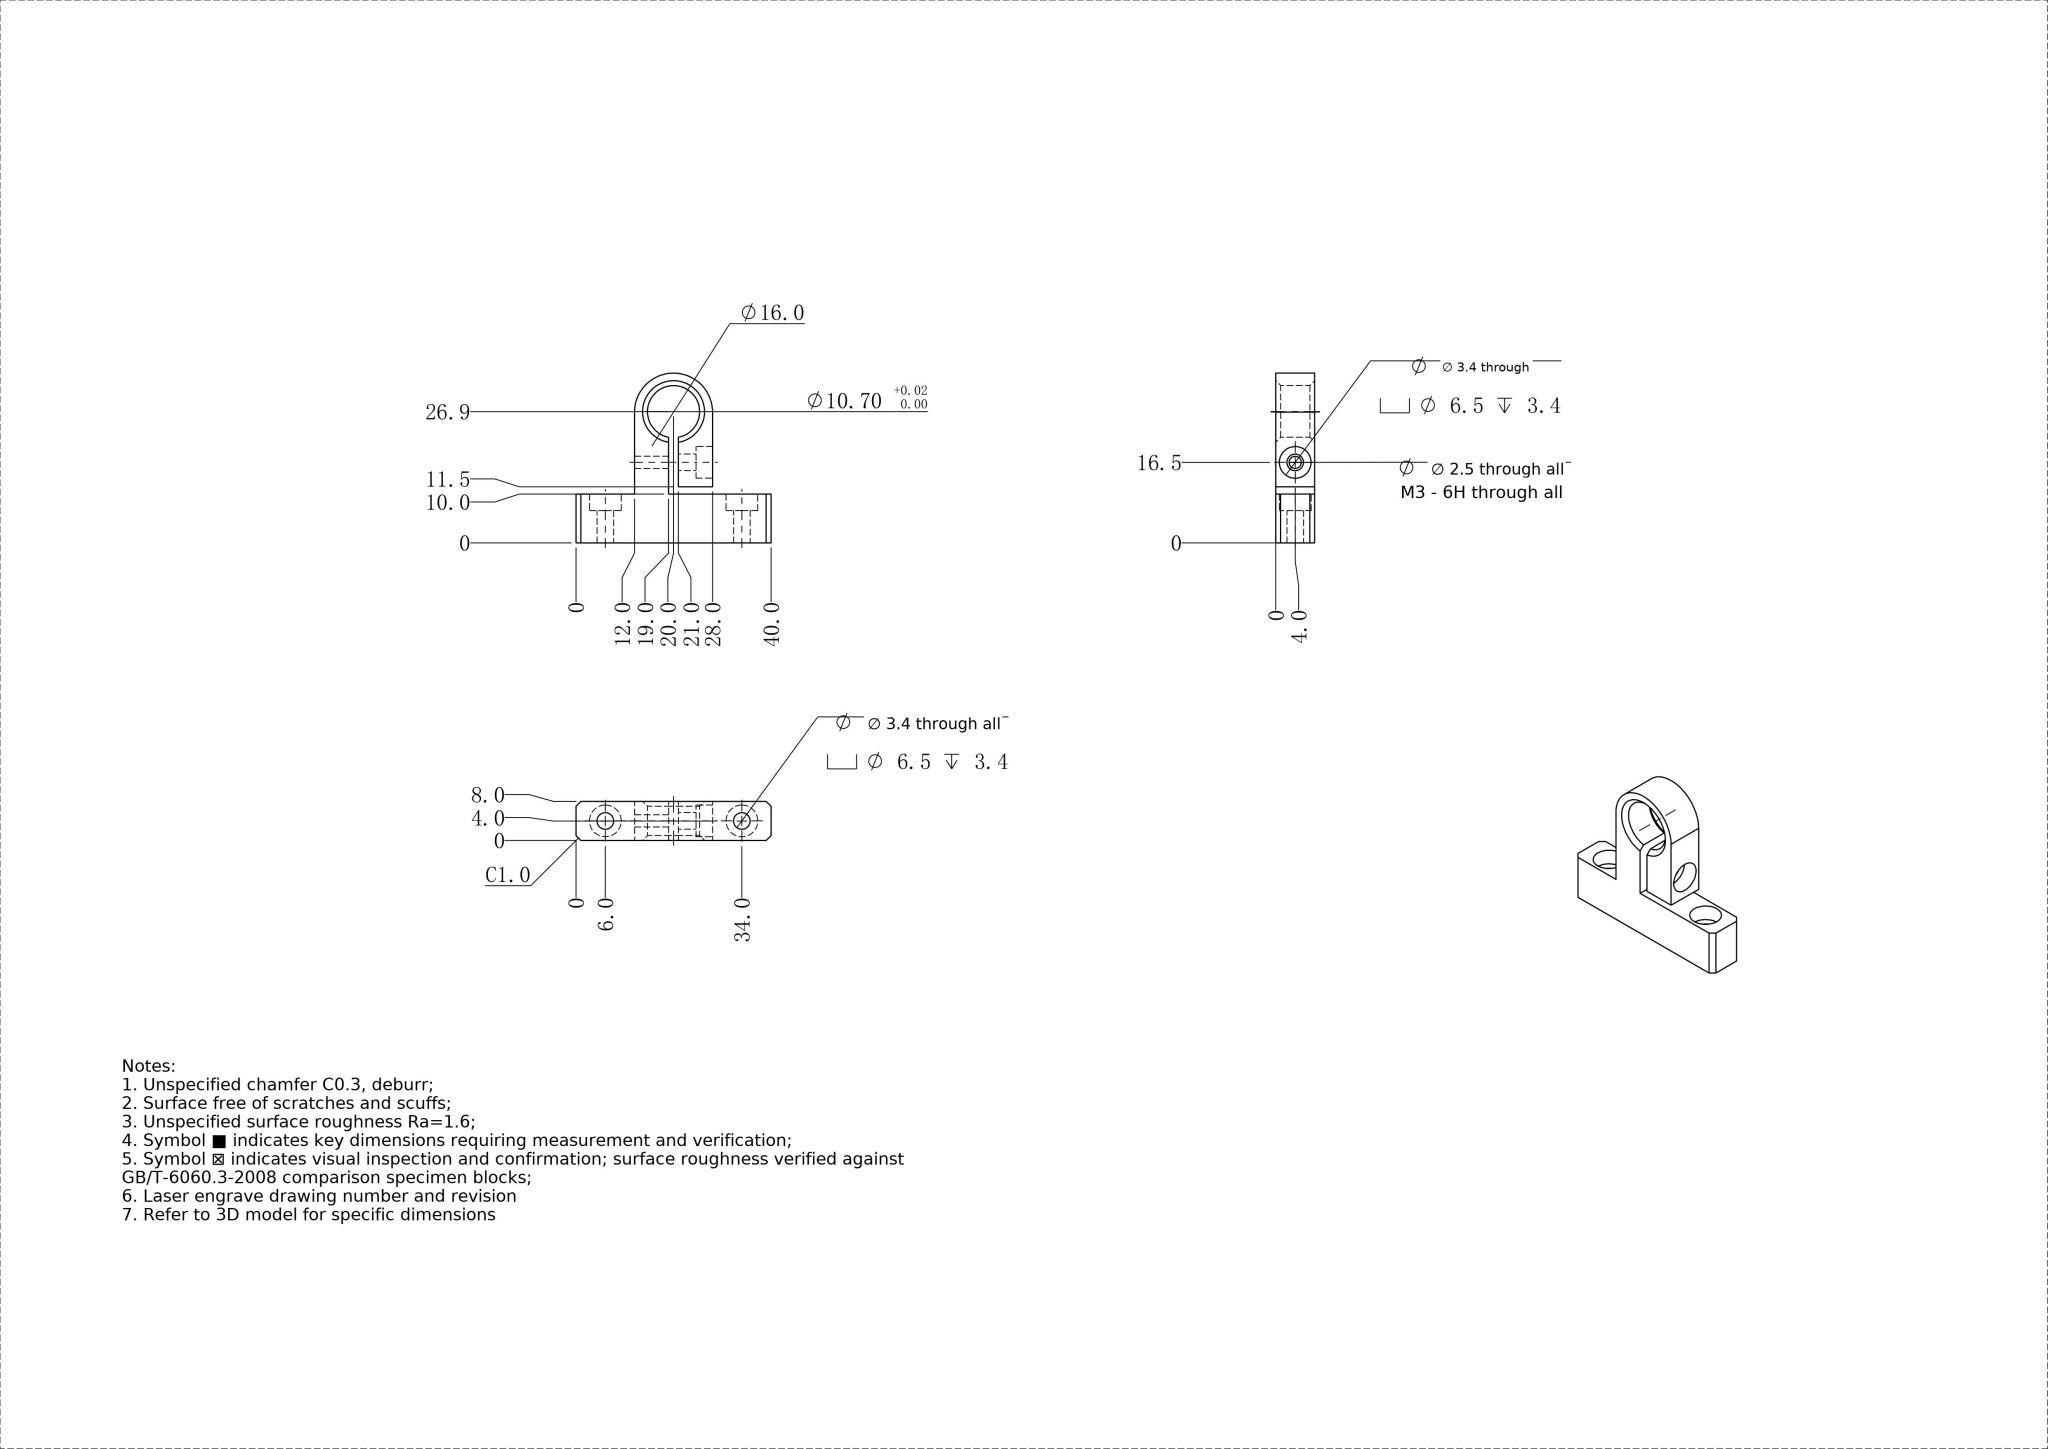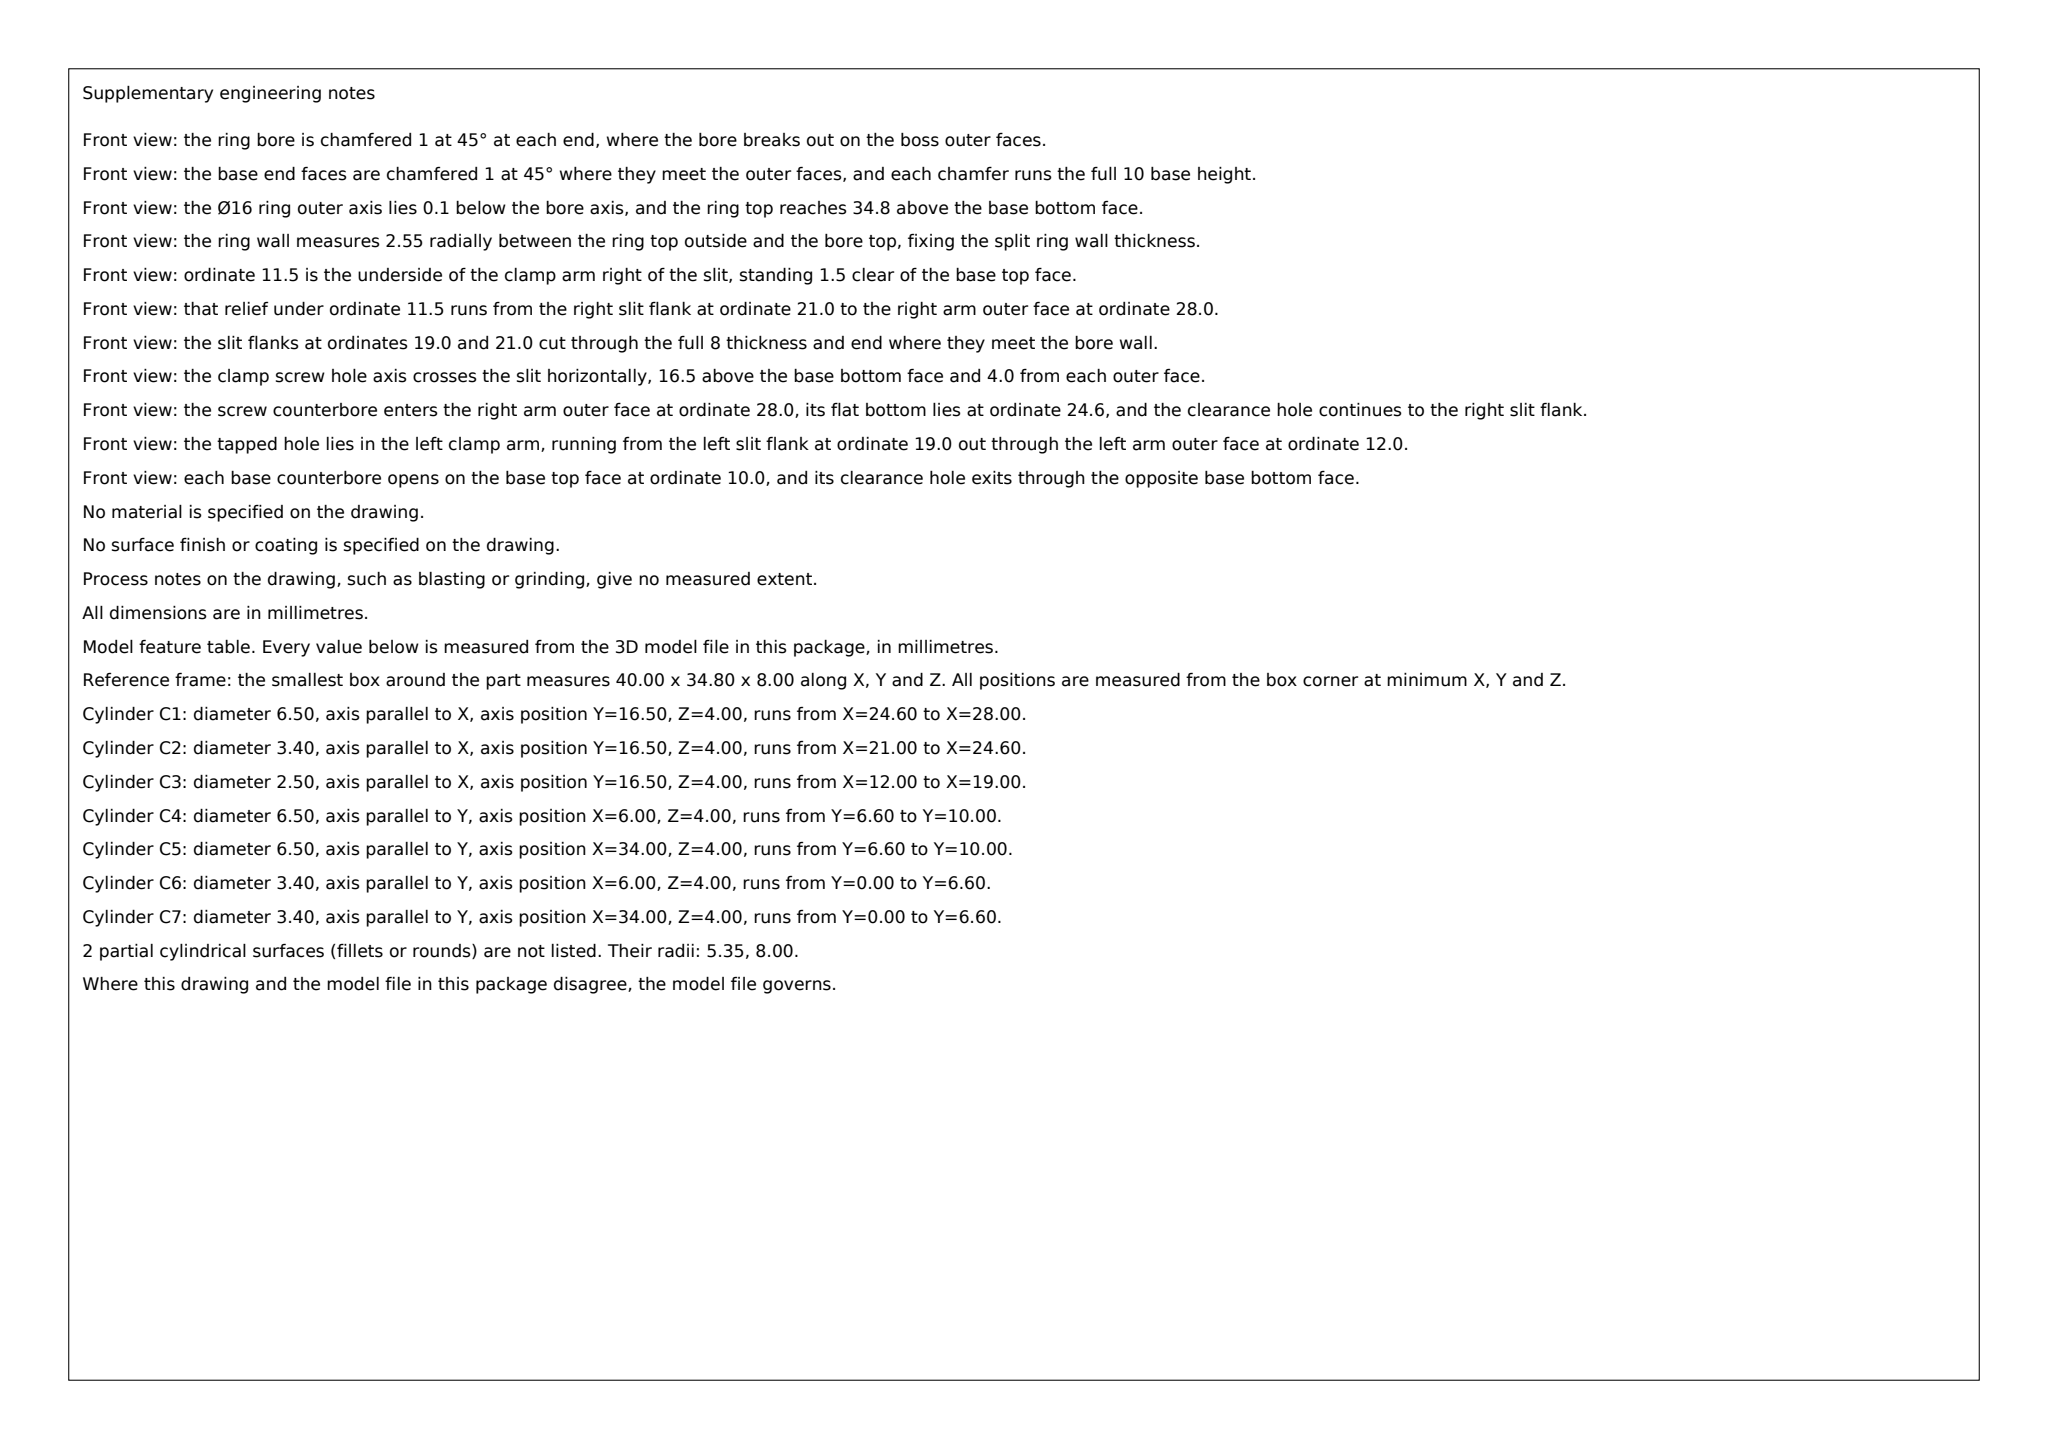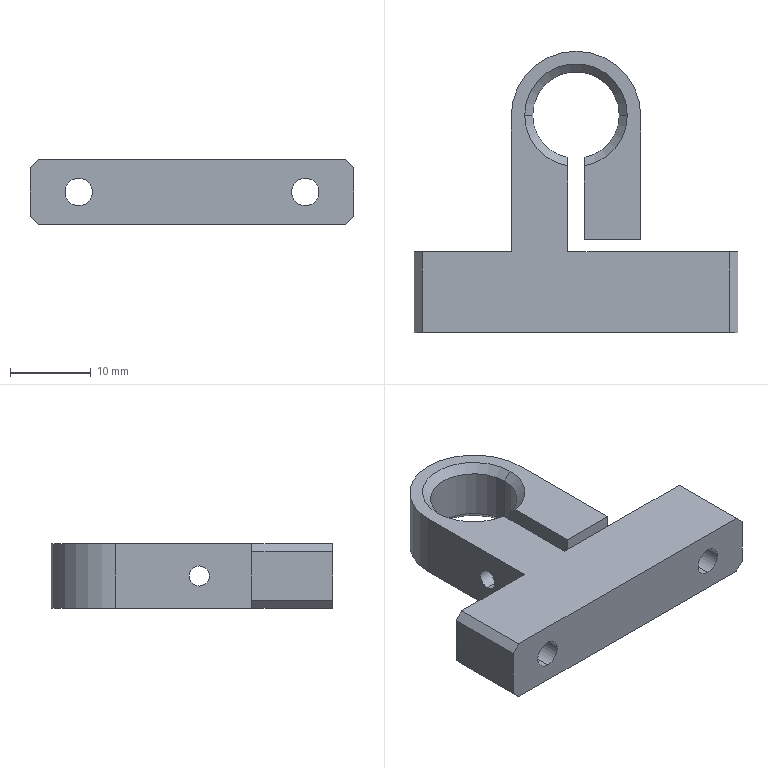Part | SolidWorks | mm | 1 solid | 43 faces | box 40 x 34.8 x 8 mm | volume 4587 mm3 | plane 19 | cylinder 18 | cone 6 | commonest cylinder face diameters 6.5 x6 3.4 x6 10.7 x3 2.5 x2 16 x1